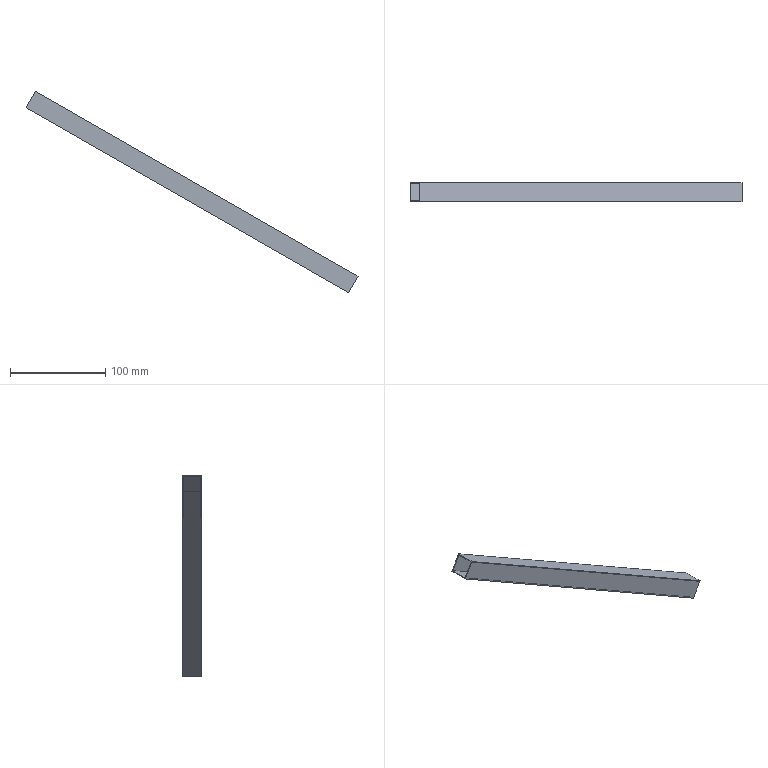Component | SolidWorks | FrontDoorFlangeWelding-2_FrontDoorRectangularTubeFrameWelding-1_390RectangularTube-1 | 1 solid | 10 faces | box 348.34 x 20 x 211.24 mm | volume 29640 mm3 | plane 10
STEP:
#1=COLOUR_RGB('',0.7922,0.8196,0.9333);
#2=FILL_AREA_STYLE_COLOUR('',#1);
#3=FILL_AREA_STYLE('',(#2));
#4=SURFACE_STYLE_FILL_AREA(#3);
#5=SURFACE_SIDE_STYLE('',(#4));
#6=SURFACE_STYLE_USAGE(.BOTH.,#5);
#7=PRESENTATION_STYLE_ASSIGNMENT((#6));
#8=CARTESIAN_POINT('',(1.249,32.011,55.374));
#9=VERTEX_POINT('',#8);
#10=CARTESIAN_POINT('',(0.8573,32.011,54.691));
#11=VERTEX_POINT('',#10);
#12=CARTESIAN_POINT('',(1.249,32.011,55.374));
#13=DIRECTION('',(-0.4971,0.,-0.8677));
#14=VECTOR('',#13,39.37);
#15=LINE('',#12,#14);
#16=EDGE_CURVE('',#9,#11,#15,.T.);
#17=ORIENTED_EDGE('',*,*,#16,.T.);
#18=CARTESIAN_POINT('',(0.8573,32.798,54.691));
#19=VERTEX_POINT('',#18);
#20=CARTESIAN_POINT('',(0.8573,32.011,54.691));
#21=DIRECTION('',(0.,1.,0.));
#22=VECTOR('',#21,39.37);
#23=LINE('',#20,#22);
#24=EDGE_CURVE('',#11,#19,#23,.T.);
#25=ORIENTED_EDGE('',*,*,#24,.T.);
#26=CARTESIAN_POINT('',(1.249,32.798,55.374));
#27=VERTEX_POINT('',#26);
#28=CARTESIAN_POINT('',(1.249,32.798,55.374));
#29=DIRECTION('',(0.4971,-0.,0.8677));
#30=VECTOR('',#29,39.37);
#31=LINE('',#28,#30);
#32=EDGE_CURVE('',#19,#27,#31,.T.);
#33=ORIENTED_EDGE('',*,*,#32,.T.);
#34=CARTESIAN_POINT('',(1.249,32.011,55.374));
#35=DIRECTION('',(-0.,-1.,-0.));
#36=VECTOR('',#35,39.37);
#37=LINE('',#34,#36);
#38=EDGE_CURVE('',#27,#9,#37,.T.);
#39=ORIENTED_EDGE('',*,*,#38,.T.);
#40=EDGE_LOOP('',(#17,#25,#33,#39));
#41=FACE_OUTER_BOUND('',#40,.T.);
#42=CARTESIAN_POINT('',(0.8769,32.05,54.725));
#43=VERTEX_POINT('',#42);
#44=CARTESIAN_POINT('',(0.8769,32.759,54.725));
#45=VERTEX_POINT('',#44);
#46=CARTESIAN_POINT('',(0.8769,32.05,54.725));
#47=DIRECTION('',(0.,1.,0.));
#48=VECTOR('',#47,39.37);
#49=LINE('',#46,#48);
#50=EDGE_CURVE('',#43,#45,#49,.T.);
#51=ORIENTED_EDGE('',*,*,#50,.F.);
#52=CARTESIAN_POINT('',(1.229,32.05,55.34));
#53=VERTEX_POINT('',#52);
#54=CARTESIAN_POINT('',(1.229,32.05,55.34));
#55=DIRECTION('',(-0.4971,0.,-0.8677));
#56=VECTOR('',#55,39.37);
#57=LINE('',#54,#56);
#58=EDGE_CURVE('',#53,#43,#57,.T.);
#59=ORIENTED_EDGE('',*,*,#58,.F.);
#60=CARTESIAN_POINT('',(1.229,32.759,55.34));
#61=VERTEX_POINT('',#60);
#62=CARTESIAN_POINT('',(1.229,32.05,55.34));
#63=DIRECTION('',(-0.,-1.,-0.));
#64=VECTOR('',#63,39.37);
#65=LINE('',#62,#64);
#66=EDGE_CURVE('',#61,#53,#65,.T.);
#67=ORIENTED_EDGE('',*,*,#66,.F.);
#68=CARTESIAN_POINT('',(1.229,32.759,55.34));
#69=DIRECTION('',(0.4971,-0.,0.8677));
#70=VECTOR('',#69,39.37);
#71=LINE('',#68,#70);
#72=EDGE_CURVE('',#45,#61,#71,.T.);
#73=ORIENTED_EDGE('',*,*,#72,.F.);
#74=EDGE_LOOP('',(#51,#59,#67,#73));
#75=FACE_BOUND('',#74,.T.);
#76=CARTESIAN_POINT('',(0.516,33.988,54.095));
#77=DIRECTION('',(0.8677,0.,-0.4971));
#78=DIRECTION('',(0.,1.,0.));
#79=AXIS2_PLACEMENT_3D('',#76,#77,#78);
#80=PLANE('',#79);
#81=ADVANCED_FACE('',(#41,#75),#80,.T.);
#82=CARTESIAN_POINT('',(-12.074,32.011,63.007));
#83=VERTEX_POINT('',#82);
#84=CARTESIAN_POINT('',(-12.465,32.011,62.324));
#85=VERTEX_POINT('',#84);
#86=CARTESIAN_POINT('',(-12.074,32.011,63.007));
#87=DIRECTION('',(-0.4971,0.,-0.8677));
#88=VECTOR('',#87,39.37);
#89=LINE('',#86,#88);
#90=EDGE_CURVE('',#83,#85,#89,.T.);
#91=ORIENTED_EDGE('',*,*,#90,.F.);
#92=CARTESIAN_POINT('',(-12.074,32.798,63.007));
#93=VERTEX_POINT('',#92);
#94=CARTESIAN_POINT('',(-12.074,32.011,63.007));
#95=DIRECTION('',(-0.,-1.,-0.));
#96=VECTOR('',#95,39.37);
#97=LINE('',#94,#96);
#98=EDGE_CURVE('',#93,#83,#97,.T.);
#99=ORIENTED_EDGE('',*,*,#98,.F.);
#100=CARTESIAN_POINT('',(-12.465,32.798,62.324));
#101=VERTEX_POINT('',#100);
#102=CARTESIAN_POINT('',(-12.074,32.798,63.007));
#103=DIRECTION('',(0.4971,-0.,0.8677));
#104=VECTOR('',#103,39.37);
#105=LINE('',#102,#104);
#106=EDGE_CURVE('',#101,#93,#105,.T.);
#107=ORIENTED_EDGE('',*,*,#106,.F.);
#108=CARTESIAN_POINT('',(-12.465,32.011,62.324));
#109=DIRECTION('',(0.,1.,0.));
#110=VECTOR('',#109,39.37);
#111=LINE('',#108,#110);
#112=EDGE_CURVE('',#85,#101,#111,.T.);
#113=ORIENTED_EDGE('',*,*,#112,.F.);
#114=EDGE_LOOP('',(#91,#99,#107,#113));
#115=FACE_OUTER_BOUND('',#114,.T.);
#116=CARTESIAN_POINT('',(-12.093,32.05,62.973));
#117=VERTEX_POINT('',#116);
#118=CARTESIAN_POINT('',(-12.446,32.05,62.358));
#119=VERTEX_POINT('',#118);
#120=CARTESIAN_POINT('',(-12.093,32.05,62.973));
#121=DIRECTION('',(-0.4971,0.,-0.8677));
#122=VECTOR('',#121,39.37);
#123=LINE('',#120,#122);
#124=EDGE_CURVE('',#117,#119,#123,.T.);
#125=ORIENTED_EDGE('',*,*,#124,.T.);
#126=CARTESIAN_POINT('',(-12.446,32.759,62.358));
#127=VERTEX_POINT('',#126);
#128=CARTESIAN_POINT('',(-12.446,32.05,62.358));
#129=DIRECTION('',(0.,1.,0.));
#130=VECTOR('',#129,39.37);
#131=LINE('',#128,#130);
#132=EDGE_CURVE('',#119,#127,#131,.T.);
#133=ORIENTED_EDGE('',*,*,#132,.T.);
#134=CARTESIAN_POINT('',(-12.093,32.759,62.973));
#135=VERTEX_POINT('',#134);
#136=CARTESIAN_POINT('',(-12.093,32.759,62.973));
#137=DIRECTION('',(0.4971,-0.,0.8677));
#138=VECTOR('',#137,39.37);
#139=LINE('',#136,#138);
#140=EDGE_CURVE('',#127,#135,#139,.T.);
#141=ORIENTED_EDGE('',*,*,#140,.T.);
#142=CARTESIAN_POINT('',(-12.093,32.05,62.973));
#143=DIRECTION('',(-0.,-1.,-0.));
#144=VECTOR('',#143,39.37);
#145=LINE('',#142,#144);
#146=EDGE_CURVE('',#135,#117,#145,.T.);
#147=ORIENTED_EDGE('',*,*,#146,.T.);
#148=EDGE_LOOP('',(#125,#133,#141,#147));
#149=FACE_BOUND('',#148,.T.);
#150=CARTESIAN_POINT('',(-12.807,33.988,61.729));
#151=DIRECTION('',(0.8677,0.,-0.4971));
#152=DIRECTION('',(0.,1.,0.));
#153=AXIS2_PLACEMENT_3D('',#150,#151,#152);
#154=PLANE('',#153);
#155=ADVANCED_FACE('',(#115,#149),#154,.F.);
#156=ORIENTED_EDGE('',*,*,#90,.T.);
#157=CARTESIAN_POINT('',(0.8573,32.011,54.691));
#158=DIRECTION('',(-0.8677,-0.,0.4971));
#159=VECTOR('',#158,39.37);
#160=LINE('',#157,#159);
#161=EDGE_CURVE('',#11,#85,#160,.T.);
#162=ORIENTED_EDGE('',*,*,#161,.F.);
#163=ORIENTED_EDGE('',*,*,#16,.F.);
#164=CARTESIAN_POINT('',(1.249,32.011,55.374));
#165=DIRECTION('',(-0.8677,-0.,0.4971));
#166=VECTOR('',#165,39.37);
#167=LINE('',#164,#166);
#168=EDGE_CURVE('',#9,#83,#167,.T.);
#169=ORIENTED_EDGE('',*,*,#168,.T.);
#170=EDGE_LOOP('',(#156,#162,#163,#169));
#171=FACE_OUTER_BOUND('',#170,.T.);
#172=CARTESIAN_POINT('',(1.249,32.011,55.374));
#173=DIRECTION('',(0.,1.,0.));
#174=DIRECTION('',(0.4971,-0.,0.8677));
#175=AXIS2_PLACEMENT_3D('',#172,#173,#174);
#176=PLANE('',#175);
#177=ADVANCED_FACE('',(#171),#176,.F.);
#178=ORIENTED_EDGE('',*,*,#112,.T.);
#179=CARTESIAN_POINT('',(0.8573,32.798,54.691));
#180=DIRECTION('',(-0.8677,-0.,0.4971));
#181=VECTOR('',#180,39.37);
#182=LINE('',#179,#181);
#183=EDGE_CURVE('',#19,#101,#182,.T.);
#184=ORIENTED_EDGE('',*,*,#183,.F.);
#185=ORIENTED_EDGE('',*,*,#24,.F.);
#186=ORIENTED_EDGE('',*,*,#161,.T.);
#187=EDGE_LOOP('',(#178,#184,#185,#186));
#188=FACE_OUTER_BOUND('',#187,.T.);
#189=CARTESIAN_POINT('',(0.8573,32.011,54.691));
#190=DIRECTION('',(0.4971,-0.,0.8677));
#191=DIRECTION('',(0.8677,0.,-0.4971));
#192=AXIS2_PLACEMENT_3D('',#189,#190,#191);
#193=PLANE('',#192);
#194=ADVANCED_FACE('',(#188),#193,.F.);
#195=ORIENTED_EDGE('',*,*,#106,.T.);
#196=CARTESIAN_POINT('',(1.249,32.798,55.374));
#197=DIRECTION('',(-0.8677,-0.,0.4971));
#198=VECTOR('',#197,39.37);
#199=LINE('',#196,#198);
#200=EDGE_CURVE('',#27,#93,#199,.T.);
#201=ORIENTED_EDGE('',*,*,#200,.F.);
#202=ORIENTED_EDGE('',*,*,#32,.F.);
#203=ORIENTED_EDGE('',*,*,#183,.T.);
#204=EDGE_LOOP('',(#195,#201,#202,#203));
#205=FACE_OUTER_BOUND('',#204,.T.);
#206=CARTESIAN_POINT('',(1.249,32.798,55.374));
#207=DIRECTION('',(-0.,-1.,-0.));
#208=DIRECTION('',(-0.4971,0.,-0.8677));
#209=AXIS2_PLACEMENT_3D('',#206,#207,#208);
#210=PLANE('',#209);
#211=ADVANCED_FACE('',(#205),#210,.F.);
#212=ORIENTED_EDGE('',*,*,#98,.T.);
#213=ORIENTED_EDGE('',*,*,#168,.F.);
#214=ORIENTED_EDGE('',*,*,#38,.F.);
#215=ORIENTED_EDGE('',*,*,#200,.T.);
#216=EDGE_LOOP('',(#212,#213,#214,#215));
#217=FACE_OUTER_BOUND('',#216,.T.);
#218=CARTESIAN_POINT('',(1.249,32.011,55.374));
#219=DIRECTION('',(-0.4971,0.,-0.8677));
#220=DIRECTION('',(-0.8677,-0.,0.4971));
#221=AXIS2_PLACEMENT_3D('',#218,#219,#220);
#222=PLANE('',#221);
#223=ADVANCED_FACE('',(#217),#222,.F.);
#224=ORIENTED_EDGE('',*,*,#124,.F.);
#225=CARTESIAN_POINT('',(1.229,32.05,55.34));
#226=DIRECTION('',(-0.8677,-0.,0.4971));
#227=VECTOR('',#226,39.37);
#228=LINE('',#225,#227);
#229=EDGE_CURVE('',#53,#117,#228,.T.);
#230=ORIENTED_EDGE('',*,*,#229,.F.);
#231=ORIENTED_EDGE('',*,*,#58,.T.);
#232=CARTESIAN_POINT('',(0.8769,32.05,54.725));
#233=DIRECTION('',(-0.8677,-0.,0.4971));
#234=VECTOR('',#233,39.37);
#235=LINE('',#232,#234);
#236=EDGE_CURVE('',#43,#119,#235,.T.);
#237=ORIENTED_EDGE('',*,*,#236,.T.);
#238=EDGE_LOOP('',(#224,#230,#231,#237));
#239=FACE_OUTER_BOUND('',#238,.T.);
#240=CARTESIAN_POINT('',(1.229,32.05,55.34));
#241=DIRECTION('',(-0.,1.,0.));
#242=DIRECTION('',(-0.8677,-0.,0.4971));
#243=AXIS2_PLACEMENT_3D('',#240,#241,#242);
#244=PLANE('',#243);
#245=ADVANCED_FACE('',(#239),#244,.T.);
#246=ORIENTED_EDGE('',*,*,#132,.F.);
#247=ORIENTED_EDGE('',*,*,#236,.F.);
#248=ORIENTED_EDGE('',*,*,#50,.T.);
#249=CARTESIAN_POINT('',(0.8769,32.759,54.725));
#250=DIRECTION('',(-0.8677,-0.,0.4971));
#251=VECTOR('',#250,39.37);
#252=LINE('',#249,#251);
#253=EDGE_CURVE('',#45,#127,#252,.T.);
#254=ORIENTED_EDGE('',*,*,#253,.T.);
#255=EDGE_LOOP('',(#246,#247,#248,#254));
#256=FACE_OUTER_BOUND('',#255,.T.);
#257=CARTESIAN_POINT('',(0.8769,32.05,54.725));
#258=DIRECTION('',(0.4971,-0.,0.8677));
#259=DIRECTION('',(0.8677,0.,-0.4971));
#260=AXIS2_PLACEMENT_3D('',#257,#258,#259);
#261=PLANE('',#260);
#262=ADVANCED_FACE('',(#256),#261,.T.);
#263=ORIENTED_EDGE('',*,*,#140,.F.);
#264=ORIENTED_EDGE('',*,*,#253,.F.);
#265=ORIENTED_EDGE('',*,*,#72,.T.);
#266=CARTESIAN_POINT('',(1.229,32.759,55.34));
#267=DIRECTION('',(-0.8677,-0.,0.4971));
#268=VECTOR('',#267,39.37);
#269=LINE('',#266,#268);
#270=EDGE_CURVE('',#61,#135,#269,.T.);
#271=ORIENTED_EDGE('',*,*,#270,.T.);
#272=EDGE_LOOP('',(#263,#264,#265,#271));
#273=FACE_OUTER_BOUND('',#272,.T.);
#274=CARTESIAN_POINT('',(1.229,32.759,55.34));
#275=DIRECTION('',(0.,-1.,-0.));
#276=DIRECTION('',(0.8677,0.,-0.4971));
#277=AXIS2_PLACEMENT_3D('',#274,#275,#276);
#278=PLANE('',#277);
#279=ADVANCED_FACE('',(#273),#278,.T.);
#280=ORIENTED_EDGE('',*,*,#146,.F.);
#281=ORIENTED_EDGE('',*,*,#270,.F.);
#282=ORIENTED_EDGE('',*,*,#66,.T.);
#283=ORIENTED_EDGE('',*,*,#229,.T.);
#284=EDGE_LOOP('',(#280,#281,#282,#283));
#285=FACE_OUTER_BOUND('',#284,.T.);
#286=CARTESIAN_POINT('',(1.229,32.05,55.34));
#287=DIRECTION('',(-0.4971,0.,-0.8677));
#288=DIRECTION('',(-0.8677,-0.,0.4971));
#289=AXIS2_PLACEMENT_3D('',#286,#287,#288);
#290=PLANE('',#289);
#291=ADVANCED_FACE('',(#285),#290,.T.);
#292=CLOSED_SHELL('',(#81,#155,#177,#194,#211,#223,#245,#262,#279,#291));
#293=MANIFOLD_SOLID_BREP('',#292);
#294=STYLED_ITEM('',(#7),#293);
#295=(LENGTH_UNIT()NAMED_UNIT(*)SI_UNIT($,.METRE.));
#296=LENGTH_MEASURE_WITH_UNIT(LENGTH_MEASURE(0.0254),#295);
#297=DIMENSIONAL_EXPONENTS(1.,0.,0.,0.,0.,0.,0.);
#298=(CONVERSION_BASED_UNIT('',#296)LENGTH_UNIT()NAMED_UNIT(#297));
#299=UNCERTAINTY_MEASURE_WITH_UNIT(LENGTH_MEASURE(0.00001),#298,'','');
#300=(NAMED_UNIT(*)PLANE_ANGLE_UNIT()SI_UNIT($,.RADIAN.));
#301=(NAMED_UNIT(*)SI_UNIT($,.STERADIAN.)SOLID_ANGLE_UNIT());
#302=(GEOMETRIC_REPRESENTATION_CONTEXT(3)GLOBAL_UNCERTAINTY_ASSIGNED_CONTEXT((#299))GLOBAL_UNIT_ASSIGNED_CONTEXT((#298,#300,#301))REPRESENTATION_CONTEXT('',''));
#303=MECHANICAL_DESIGN_GEOMETRIC_PRESENTATION_REPRESENTATION('',(#294),#302);
#304=PRESENTATION_LAYER_ASSIGNMENT('','',(#294));
#305=CARTESIAN_POINT('',(0.,0.,0.));
#306=DIRECTION('',(0.,0.,1.));
#307=DIRECTION('',(1.,0.,0.));
#308=AXIS2_PLACEMENT_3D('',#305,#306,#307);
#309=(LENGTH_UNIT()NAMED_UNIT(*)SI_UNIT($,.METRE.));
#310=LENGTH_MEASURE_WITH_UNIT(LENGTH_MEASURE(0.0254),#309);
#311=DIMENSIONAL_EXPONENTS(1.,0.,0.,0.,0.,0.,0.);
#312=(CONVERSION_BASED_UNIT('',#310)LENGTH_UNIT()NAMED_UNIT(#311));
#313=UNCERTAINTY_MEASURE_WITH_UNIT(LENGTH_MEASURE(0.00001),#312,'','');
#314=(NAMED_UNIT(*)PLANE_ANGLE_UNIT()SI_UNIT($,.RADIAN.));
#315=(NAMED_UNIT(*)SI_UNIT($,.STERADIAN.)SOLID_ANGLE_UNIT());
#316=(GEOMETRIC_REPRESENTATION_CONTEXT(3)GLOBAL_UNCERTAINTY_ASSIGNED_CONTEXT((#313))GLOBAL_UNIT_ASSIGNED_CONTEXT((#312,#314,#315))REPRESENTATION_CONTEXT('',''));
#317=ADVANCED_BREP_SHAPE_REPRESENTATION('',(#293,#308),#316);